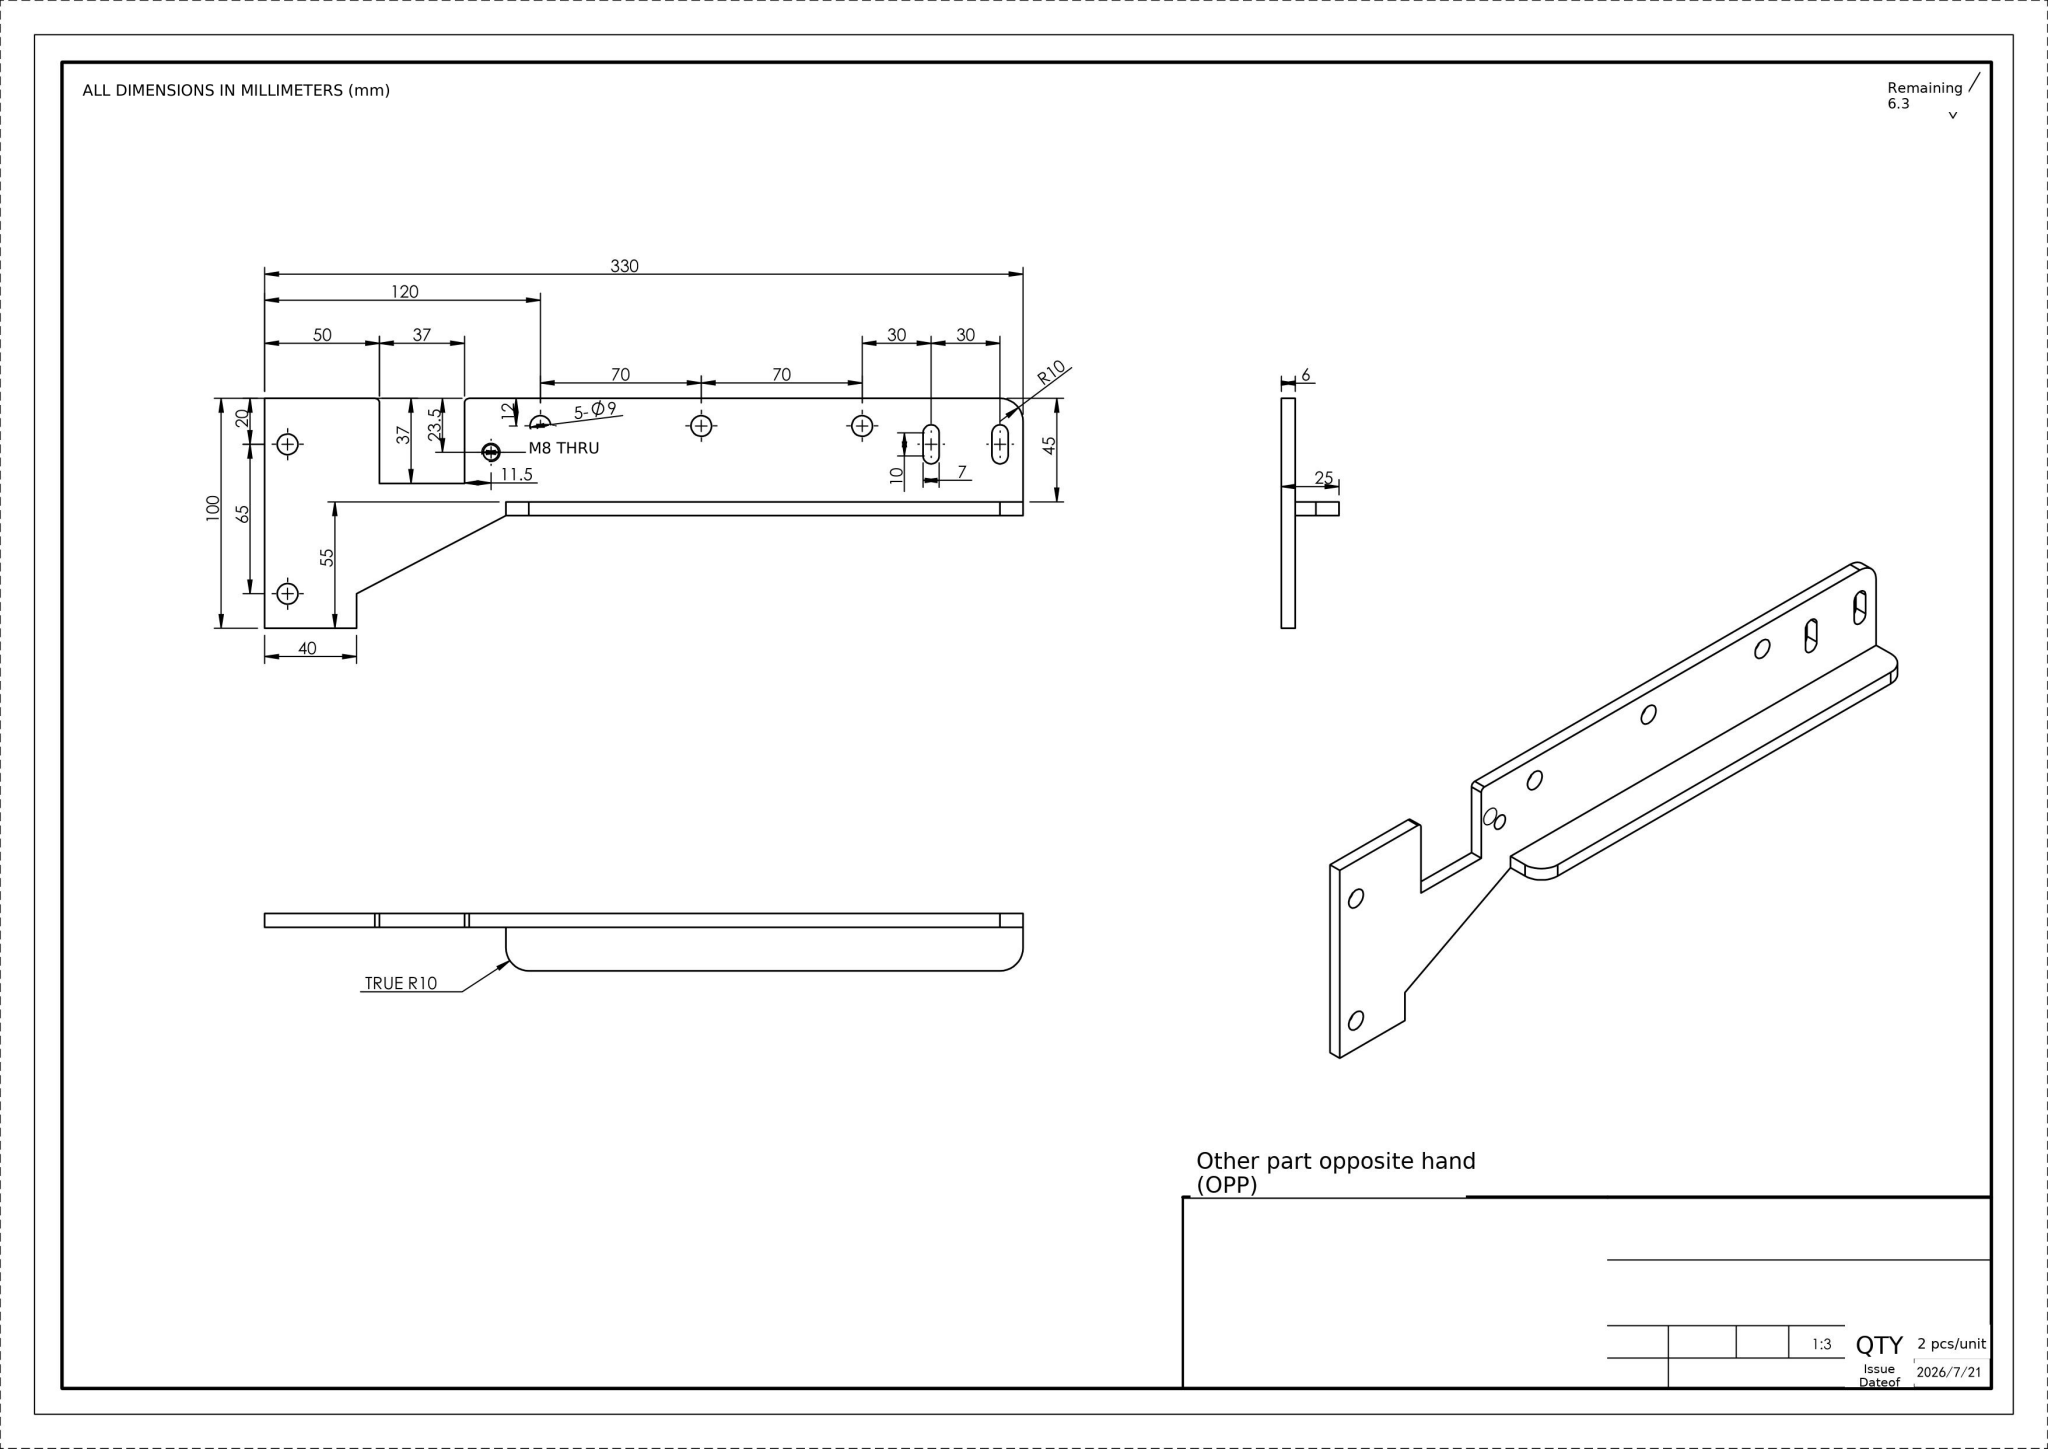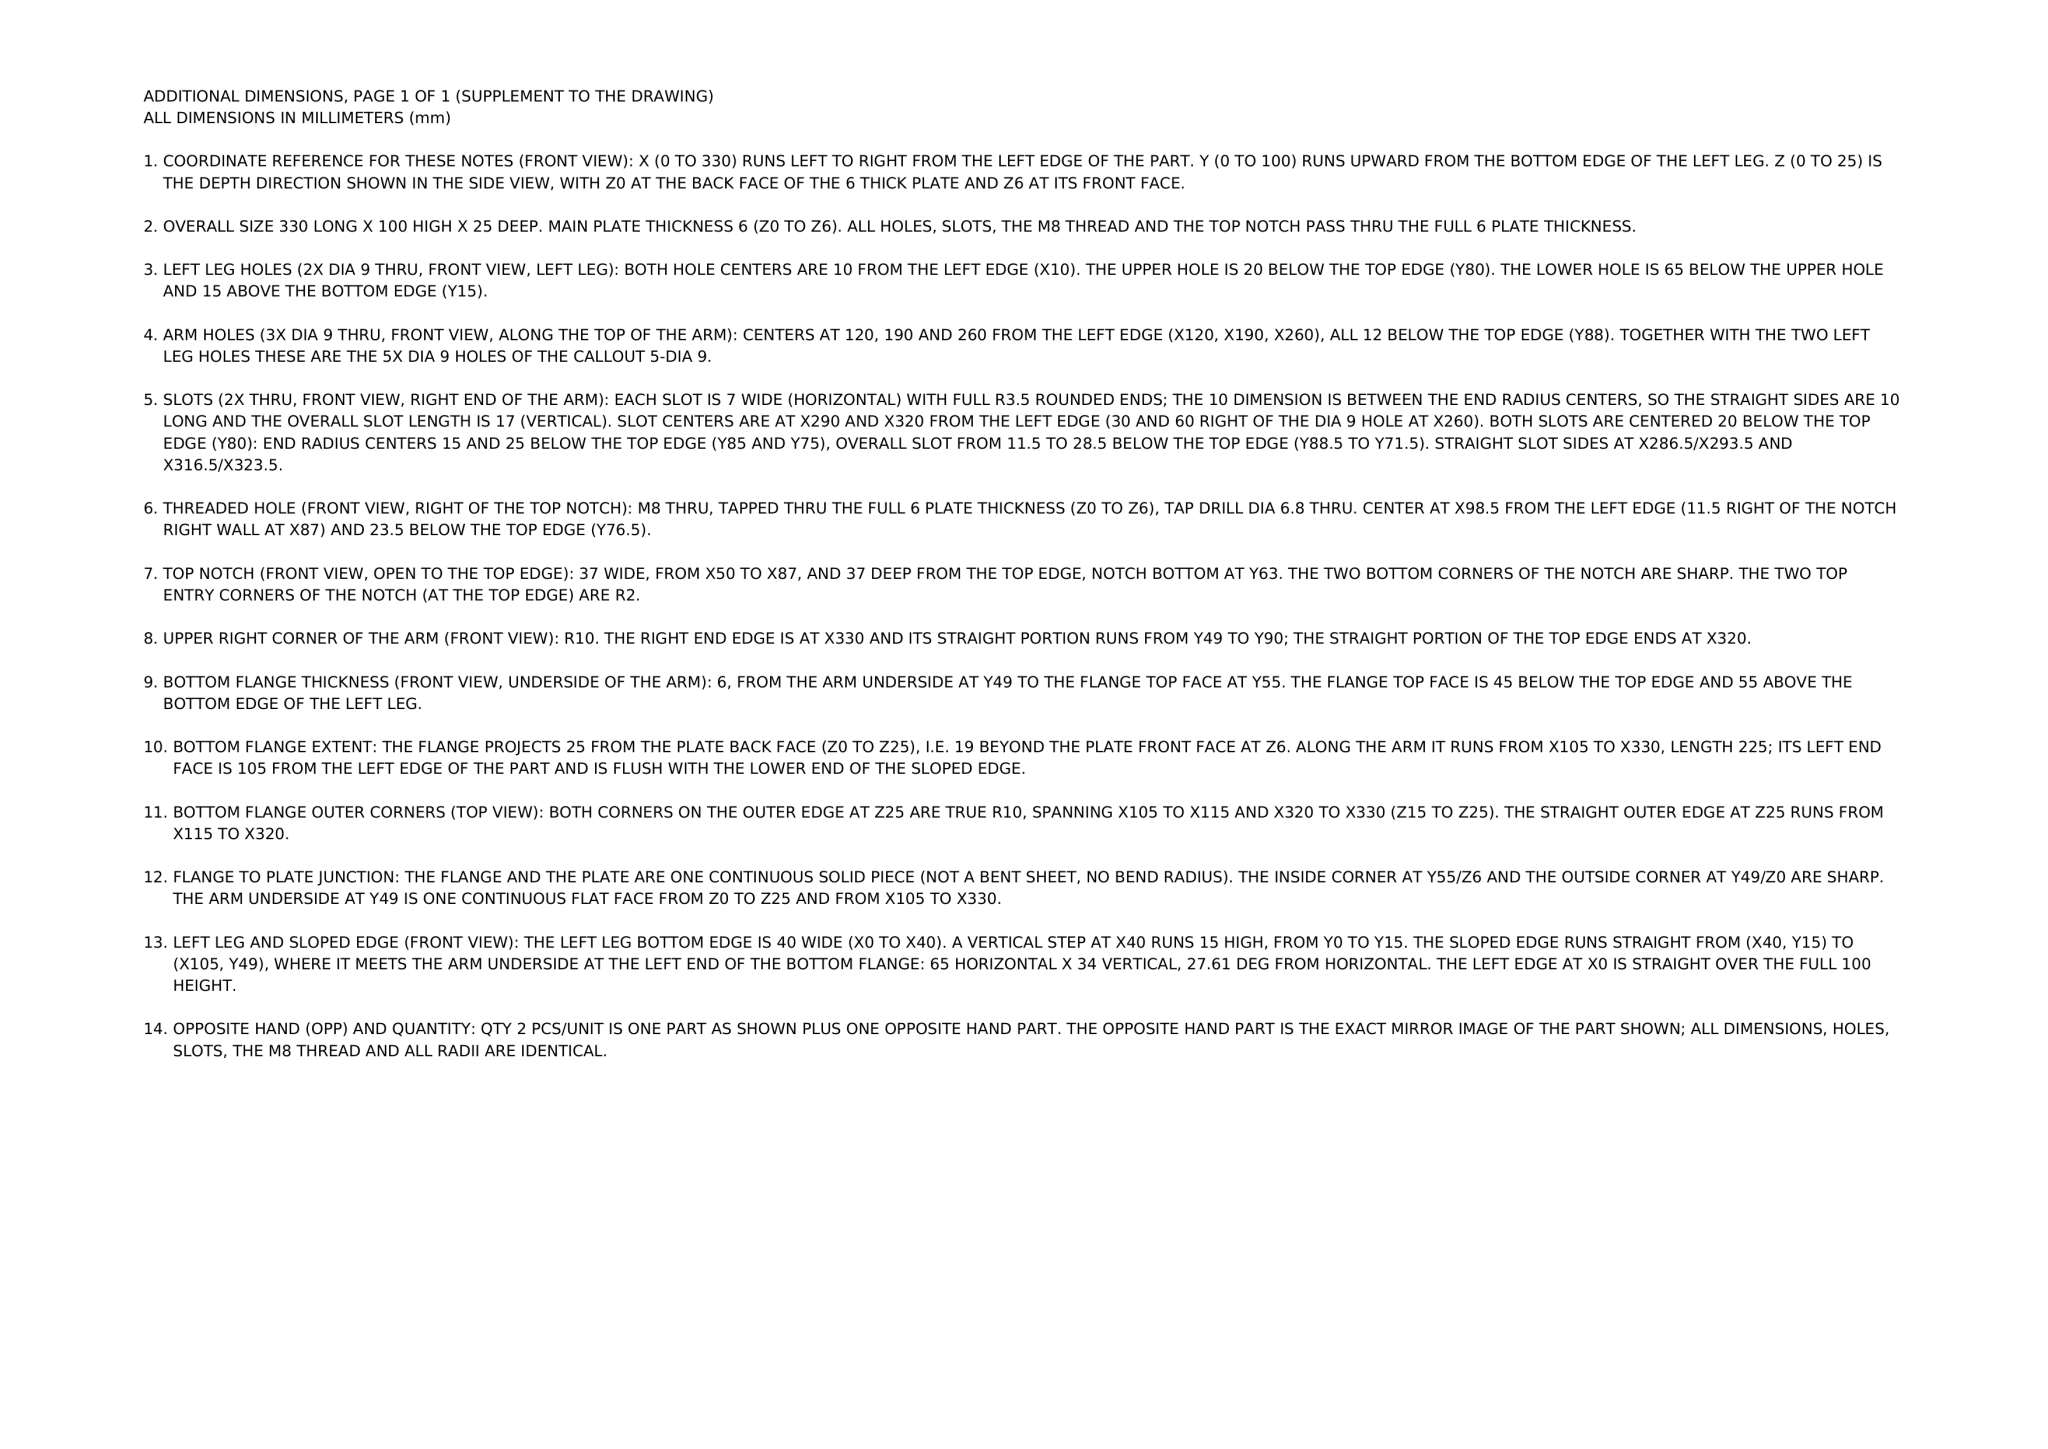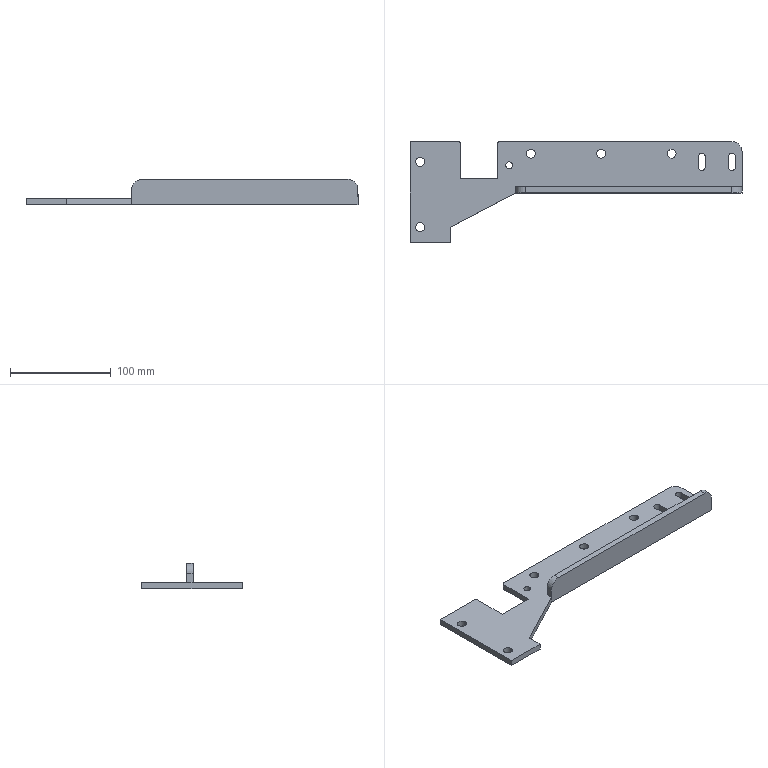Part | NX | mm | 1 solid | 41 faces | box 330 x 100 x 25 mm | volume 132981 mm3 | cylinder 21 | plane 20 | commonest cylinder face diameters 9 x10 7 x4 20 x3 6.8 x2 4 x2